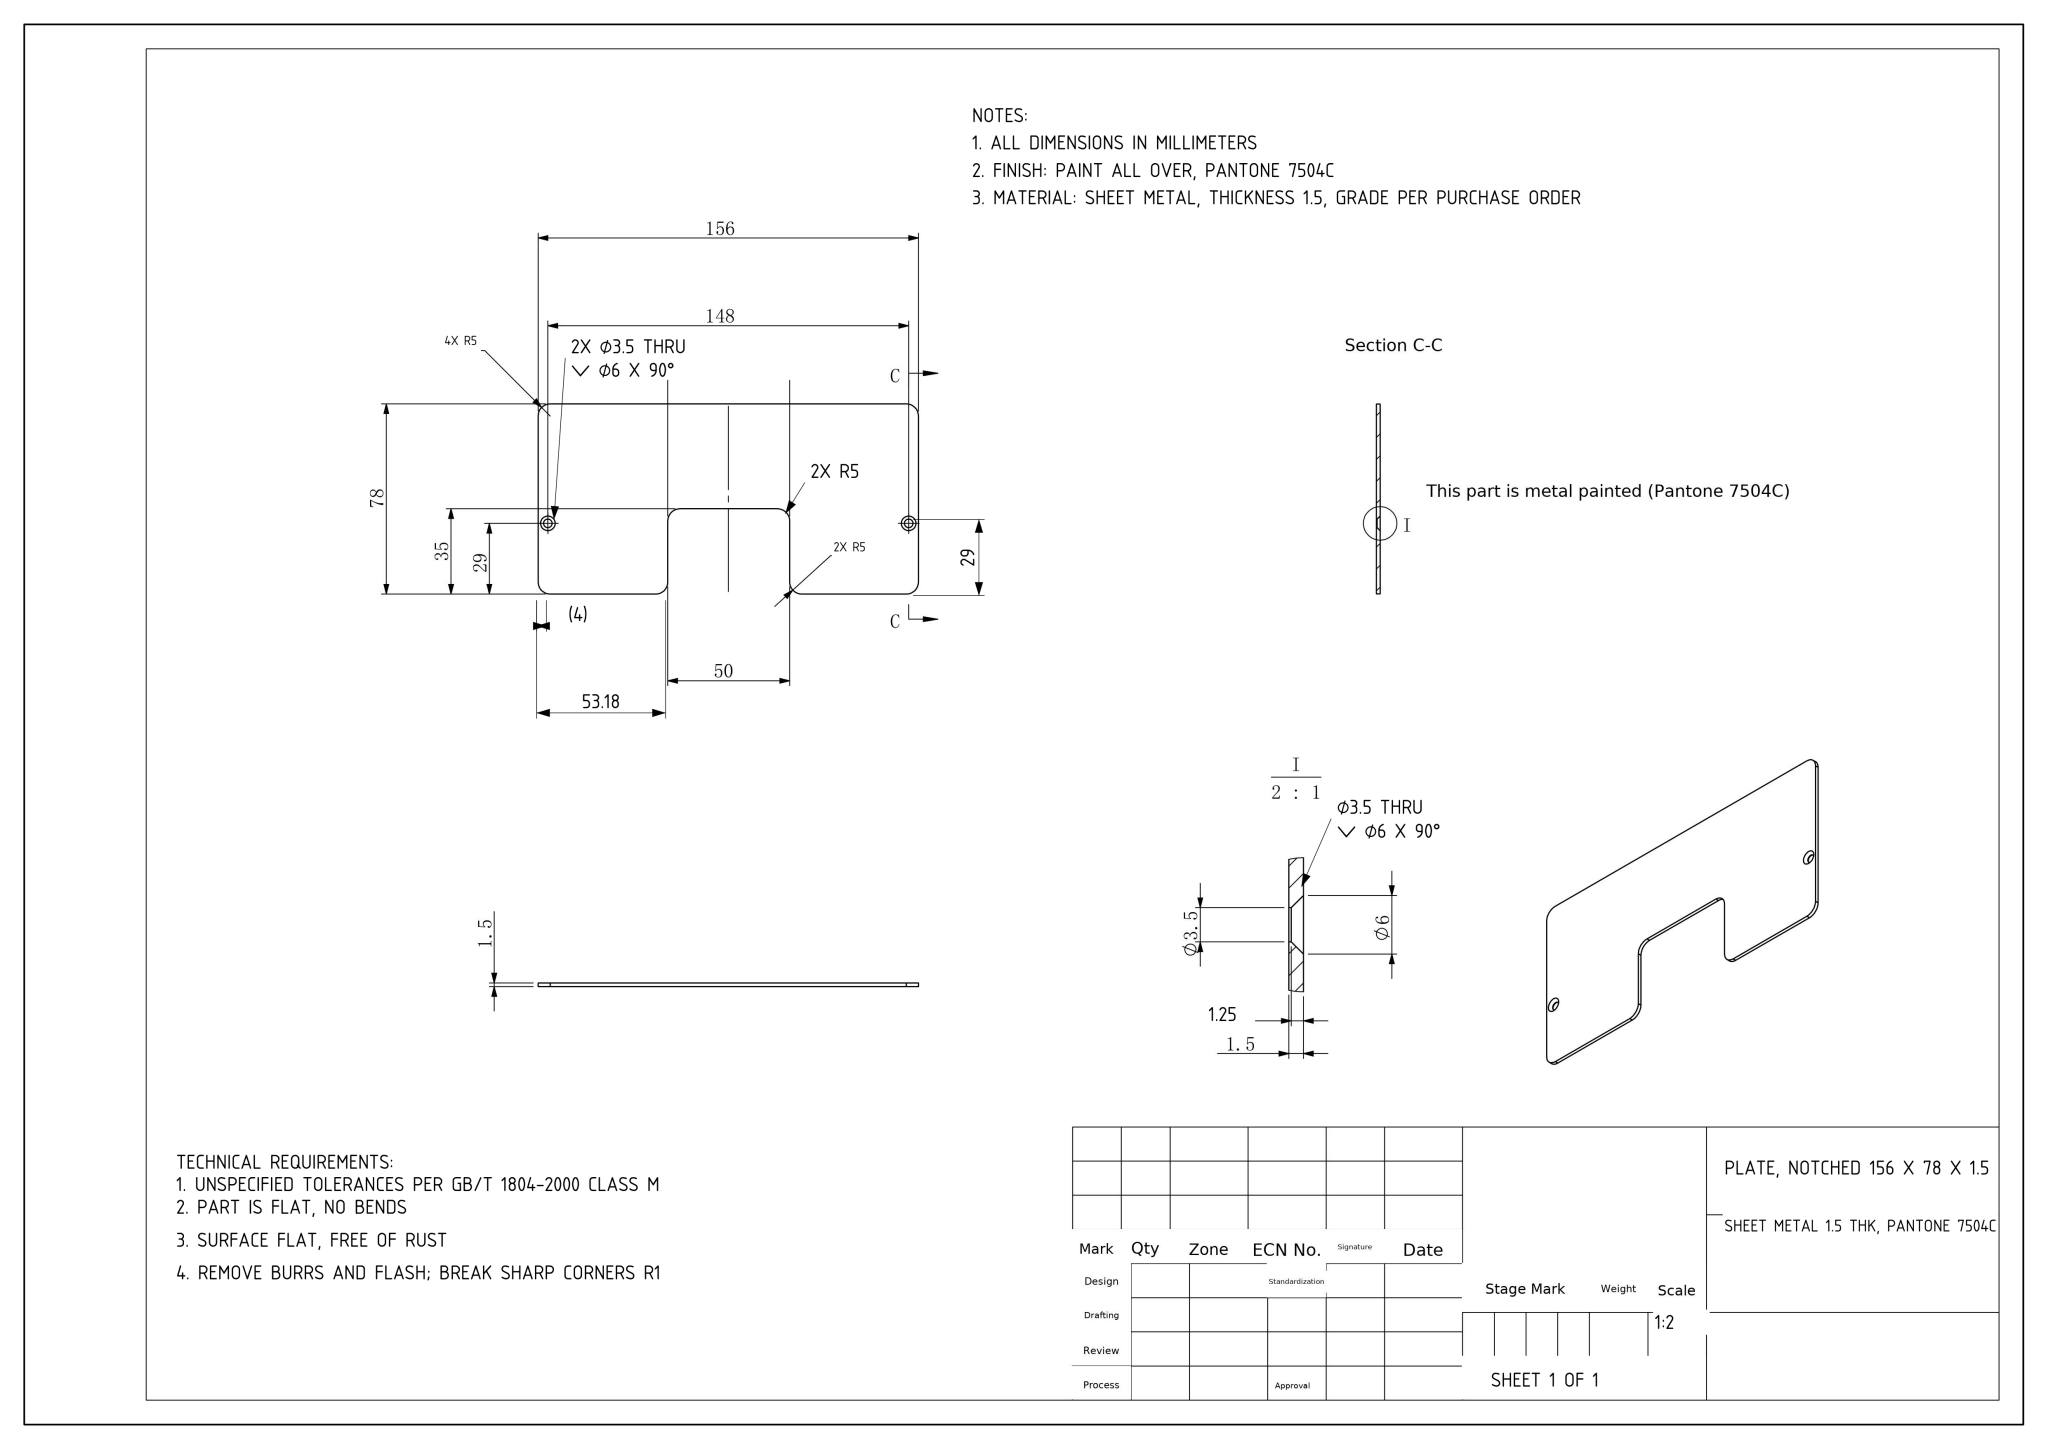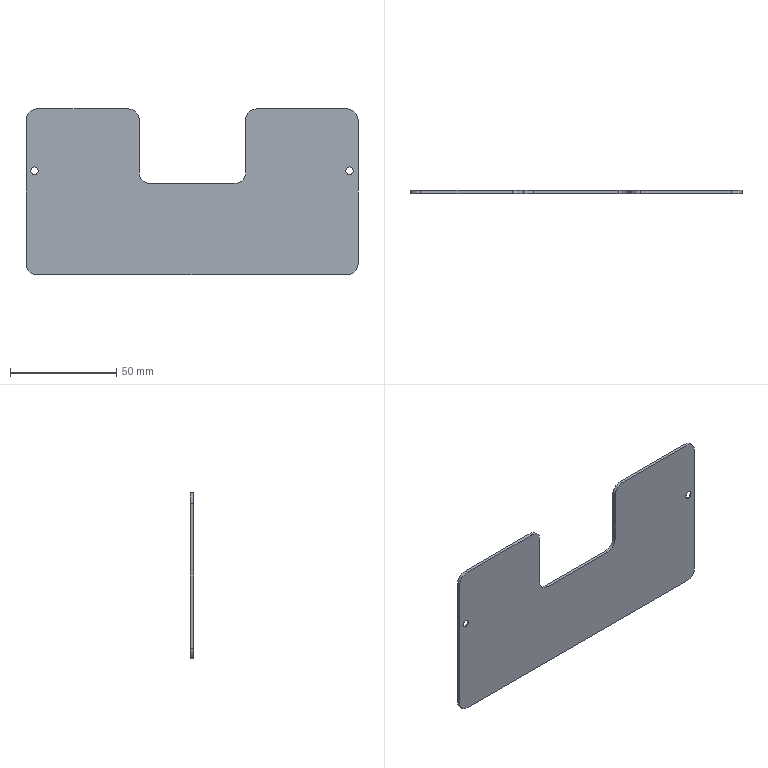Part | NX | mm | 1 solid | 26 faces | box 156 x 1.5 x 78 mm | volume 15545 mm3 | cylinder 12 | plane 10 | cone 4 | commonest cylinder face diameters 10 x8 3.5 x4
STEP:
#1=COLOUR_RGB('',0.7529,0.7529,0.7529);
#2=FILL_AREA_STYLE_COLOUR('',#1);
#3=FILL_AREA_STYLE('',(#2));
#4=SURFACE_STYLE_FILL_AREA(#3);
#5=SURFACE_SIDE_STYLE('',(#4));
#6=SURFACE_STYLE_USAGE(.BOTH.,#5);
#7=PRESENTATION_STYLE_ASSIGNMENT((#6));
#8=CARTESIAN_POINT('',(74.,-1.25,8.));
#9=VERTEX_POINT('',#8);
#10=CARTESIAN_POINT('',(74.,-1.25,11.5));
#11=VERTEX_POINT('',#10);
#12=CARTESIAN_POINT('',(74.,-1.25,9.75));
#13=DIRECTION('',(0.,1.,0.));
#14=DIRECTION('',(0.,0.,1.));
#15=AXIS2_PLACEMENT_3D('',#12,#13,#14);
#16=CIRCLE('',#15,1.75);
#17=EDGE_CURVE('',#9,#11,#16,.T.);
#18=ORIENTED_EDGE('',*,*,#17,.F.);
#19=CARTESIAN_POINT('',(74.,0.,6.75));
#20=VERTEX_POINT('',#19);
#21=CARTESIAN_POINT('',(74.,0.,6.75));
#22=DIRECTION('',(0.,0.7071,-0.7071));
#23=VECTOR('',#22,1000.);
#24=LINE('',#21,#23);
#25=EDGE_CURVE('',#9,#20,#24,.T.);
#26=ORIENTED_EDGE('',*,*,#25,.T.);
#27=CARTESIAN_POINT('',(74.,0.,12.75));
#28=VERTEX_POINT('',#27);
#29=CARTESIAN_POINT('',(74.,0.,9.75));
#30=DIRECTION('',(0.,-1.,0.));
#31=DIRECTION('',(0.,0.,1.));
#32=AXIS2_PLACEMENT_3D('',#29,#30,#31);
#33=CIRCLE('',#32,3.);
#34=EDGE_CURVE('',#28,#20,#33,.T.);
#35=ORIENTED_EDGE('',*,*,#34,.F.);
#36=CARTESIAN_POINT('',(74.,0.,12.75));
#37=DIRECTION('',(0.,0.7071,0.7071));
#38=VECTOR('',#37,1000.);
#39=LINE('',#36,#38);
#40=EDGE_CURVE('',#11,#28,#39,.T.);
#41=ORIENTED_EDGE('',*,*,#40,.F.);
#42=EDGE_LOOP('',(#18,#26,#35,#41));
#43=FACE_OUTER_BOUND('',#42,.T.);
#44=CARTESIAN_POINT('',(74.,0.,9.75));
#45=DIRECTION('',(0.,1.,0.));
#46=DIRECTION('',(0.,0.,1.));
#47=AXIS2_PLACEMENT_3D('',#44,#45,#46);
#48=CONICAL_SURFACE('',#47,3.,0.7854);
#49=ADVANCED_FACE('',(#43),#48,.F.);
#50=CARTESIAN_POINT('',(-74.,-1.25,8.));
#51=VERTEX_POINT('',#50);
#52=CARTESIAN_POINT('',(-74.,-1.25,11.5));
#53=VERTEX_POINT('',#52);
#54=CARTESIAN_POINT('',(-74.,-1.25,9.75));
#55=DIRECTION('',(0.,1.,0.));
#56=DIRECTION('',(0.,0.,1.));
#57=AXIS2_PLACEMENT_3D('',#54,#55,#56);
#58=CIRCLE('',#57,1.75);
#59=EDGE_CURVE('',#51,#53,#58,.T.);
#60=ORIENTED_EDGE('',*,*,#59,.F.);
#61=CARTESIAN_POINT('',(-74.,0.,6.75));
#62=VERTEX_POINT('',#61);
#63=CARTESIAN_POINT('',(-74.,0.,6.75));
#64=DIRECTION('',(0.,0.7071,-0.7071));
#65=VECTOR('',#64,1000.);
#66=LINE('',#63,#65);
#67=EDGE_CURVE('',#51,#62,#66,.T.);
#68=ORIENTED_EDGE('',*,*,#67,.T.);
#69=CARTESIAN_POINT('',(-74.,0.,12.75));
#70=VERTEX_POINT('',#69);
#71=CARTESIAN_POINT('',(-74.,0.,9.75));
#72=DIRECTION('',(0.,-1.,0.));
#73=DIRECTION('',(0.,0.,1.));
#74=AXIS2_PLACEMENT_3D('',#71,#72,#73);
#75=CIRCLE('',#74,3.);
#76=EDGE_CURVE('',#70,#62,#75,.T.);
#77=ORIENTED_EDGE('',*,*,#76,.F.);
#78=CARTESIAN_POINT('',(-74.,0.,12.75));
#79=DIRECTION('',(0.,0.7071,0.7071));
#80=VECTOR('',#79,1000.);
#81=LINE('',#78,#80);
#82=EDGE_CURVE('',#53,#70,#81,.T.);
#83=ORIENTED_EDGE('',*,*,#82,.F.);
#84=EDGE_LOOP('',(#60,#68,#77,#83));
#85=FACE_OUTER_BOUND('',#84,.T.);
#86=CARTESIAN_POINT('',(-74.,0.,9.75));
#87=DIRECTION('',(0.,1.,0.));
#88=DIRECTION('',(0.,0.,1.));
#89=AXIS2_PLACEMENT_3D('',#86,#87,#88);
#90=CONICAL_SURFACE('',#89,3.,0.7854);
#91=ADVANCED_FACE('',(#85),#90,.F.);
#92=ORIENTED_EDGE('',*,*,#17,.T.);
#93=CARTESIAN_POINT('',(74.,-1.5,11.5));
#94=VERTEX_POINT('',#93);
#95=CARTESIAN_POINT('',(74.,55.65,11.5));
#96=DIRECTION('',(0.,-1.,0.));
#97=VECTOR('',#96,1000.);
#98=LINE('',#95,#97);
#99=EDGE_CURVE('',#11,#94,#98,.T.);
#100=ORIENTED_EDGE('',*,*,#99,.T.);
#101=CARTESIAN_POINT('',(74.,-1.5,8.));
#102=VERTEX_POINT('',#101);
#103=CARTESIAN_POINT('',(74.,-1.5,9.75));
#104=DIRECTION('',(0.,1.,0.));
#105=DIRECTION('',(1.,0.,0.));
#106=AXIS2_PLACEMENT_3D('',#103,#104,#105);
#107=CIRCLE('',#106,1.75);
#108=EDGE_CURVE('',#102,#94,#107,.T.);
#109=ORIENTED_EDGE('',*,*,#108,.F.);
#110=CARTESIAN_POINT('',(74.,55.65,8.));
#111=DIRECTION('',(0.,-1.,0.));
#112=VECTOR('',#111,1000.);
#113=LINE('',#110,#112);
#114=EDGE_CURVE('',#9,#102,#113,.T.);
#115=ORIENTED_EDGE('',*,*,#114,.F.);
#116=EDGE_LOOP('',(#92,#100,#109,#115));
#117=FACE_OUTER_BOUND('',#116,.T.);
#118=CARTESIAN_POINT('',(74.,55.65,9.75));
#119=DIRECTION('',(0.,-1.,0.));
#120=DIRECTION('',(0.,0.,-1.));
#121=AXIS2_PLACEMENT_3D('',#118,#119,#120);
#122=CYLINDRICAL_SURFACE('',#121,1.75);
#123=ADVANCED_FACE('',(#117),#122,.F.);
#124=ORIENTED_EDGE('',*,*,#59,.T.);
#125=CARTESIAN_POINT('',(-74.,-1.5,11.5));
#126=VERTEX_POINT('',#125);
#127=CARTESIAN_POINT('',(-74.,55.65,11.5));
#128=DIRECTION('',(0.,-1.,0.));
#129=VECTOR('',#128,1000.);
#130=LINE('',#127,#129);
#131=EDGE_CURVE('',#53,#126,#130,.T.);
#132=ORIENTED_EDGE('',*,*,#131,.T.);
#133=CARTESIAN_POINT('',(-74.,-1.5,8.));
#134=VERTEX_POINT('',#133);
#135=CARTESIAN_POINT('',(-74.,-1.5,9.75));
#136=DIRECTION('',(0.,1.,0.));
#137=DIRECTION('',(1.,0.,0.));
#138=AXIS2_PLACEMENT_3D('',#135,#136,#137);
#139=CIRCLE('',#138,1.75);
#140=EDGE_CURVE('',#134,#126,#139,.T.);
#141=ORIENTED_EDGE('',*,*,#140,.F.);
#142=CARTESIAN_POINT('',(-74.,55.65,8.));
#143=DIRECTION('',(0.,-1.,0.));
#144=VECTOR('',#143,1000.);
#145=LINE('',#142,#144);
#146=EDGE_CURVE('',#51,#134,#145,.T.);
#147=ORIENTED_EDGE('',*,*,#146,.F.);
#148=EDGE_LOOP('',(#124,#132,#141,#147));
#149=FACE_OUTER_BOUND('',#148,.T.);
#150=CARTESIAN_POINT('',(-74.,55.65,9.75));
#151=DIRECTION('',(0.,-1.,0.));
#152=DIRECTION('',(0.,0.,-1.));
#153=AXIS2_PLACEMENT_3D('',#150,#151,#152);
#154=CYLINDRICAL_SURFACE('',#153,1.75);
#155=ADVANCED_FACE('',(#149),#154,.F.);
#156=CARTESIAN_POINT('',(30.185,0.,38.75));
#157=VERTEX_POINT('',#156);
#158=CARTESIAN_POINT('',(73.,0.,38.75));
#159=VERTEX_POINT('',#158);
#160=CARTESIAN_POINT('',(-78.5,0.,38.75));
#161=DIRECTION('',(1.,0.,0.));
#162=VECTOR('',#161,1000.);
#163=LINE('',#160,#162);
#164=EDGE_CURVE('',#157,#159,#163,.T.);
#165=ORIENTED_EDGE('',*,*,#164,.F.);
#166=CARTESIAN_POINT('',(30.185,-1.5,38.75));
#167=VERTEX_POINT('',#166);
#168=CARTESIAN_POINT('',(30.185,0.,38.75));
#169=DIRECTION('',(0.,-1.,0.));
#170=VECTOR('',#169,1000.);
#171=LINE('',#168,#170);
#172=EDGE_CURVE('',#157,#167,#171,.T.);
#173=ORIENTED_EDGE('',*,*,#172,.T.);
#174=CARTESIAN_POINT('',(73.,-1.5,38.75));
#175=VERTEX_POINT('',#174);
#176=CARTESIAN_POINT('',(-78.5,-1.5,38.75));
#177=DIRECTION('',(1.,0.,0.));
#178=VECTOR('',#177,1000.);
#179=LINE('',#176,#178);
#180=EDGE_CURVE('',#167,#175,#179,.T.);
#181=ORIENTED_EDGE('',*,*,#180,.T.);
#182=CARTESIAN_POINT('',(73.,0.,38.75));
#183=DIRECTION('',(0.,1.,0.));
#184=VECTOR('',#183,1000.);
#185=LINE('',#182,#184);
#186=EDGE_CURVE('',#175,#159,#185,.T.);
#187=ORIENTED_EDGE('',*,*,#186,.T.);
#188=EDGE_LOOP('',(#165,#173,#181,#187));
#189=FACE_OUTER_BOUND('',#188,.T.);
#190=CARTESIAN_POINT('',(-78.5,0.,38.75));
#191=DIRECTION('',(0.,0.,1.));
#192=DIRECTION('',(1.,0.,0.));
#193=AXIS2_PLACEMENT_3D('',#190,#191,#192);
#194=PLANE('',#193);
#195=ADVANCED_FACE('',(#189),#194,.T.);
#196=ORIENTED_EDGE('',*,*,#140,.T.);
#197=CARTESIAN_POINT('',(-74.,-1.5,9.75));
#198=DIRECTION('',(0.,1.,0.));
#199=DIRECTION('',(1.,0.,0.));
#200=AXIS2_PLACEMENT_3D('',#197,#198,#199);
#201=CIRCLE('',#200,1.75);
#202=EDGE_CURVE('',#126,#134,#201,.T.);
#203=ORIENTED_EDGE('',*,*,#202,.T.);
#204=EDGE_LOOP('',(#196,#203));
#205=FACE_BOUND('',#204,.T.);
#206=CARTESIAN_POINT('',(-24.815,-1.5,8.75));
#207=VERTEX_POINT('',#206);
#208=CARTESIAN_POINT('',(-24.815,-1.5,33.75));
#209=VERTEX_POINT('',#208);
#210=CARTESIAN_POINT('',(-24.815,-1.5,39.75));
#211=DIRECTION('',(0.,0.,1.));
#212=VECTOR('',#211,1000.);
#213=LINE('',#210,#212);
#214=EDGE_CURVE('',#207,#209,#213,.T.);
#215=ORIENTED_EDGE('',*,*,#214,.T.);
#216=CARTESIAN_POINT('',(-29.815,-1.5,38.75));
#217=VERTEX_POINT('',#216);
#218=CARTESIAN_POINT('',(-29.815,-1.5,33.75));
#219=DIRECTION('',(0.,-1.,0.));
#220=DIRECTION('',(0.,0.,1.));
#221=AXIS2_PLACEMENT_3D('',#218,#219,#220);
#222=CIRCLE('',#221,5.);
#223=EDGE_CURVE('',#209,#217,#222,.T.);
#224=ORIENTED_EDGE('',*,*,#223,.T.);
#225=CARTESIAN_POINT('',(-73.,-1.5,38.75));
#226=VERTEX_POINT('',#225);
#227=CARTESIAN_POINT('',(-78.5,-1.5,38.75));
#228=DIRECTION('',(1.,0.,0.));
#229=VECTOR('',#228,1000.);
#230=LINE('',#227,#229);
#231=EDGE_CURVE('',#226,#217,#230,.T.);
#232=ORIENTED_EDGE('',*,*,#231,.F.);
#233=CARTESIAN_POINT('',(-78.,-1.5,33.75));
#234=VERTEX_POINT('',#233);
#235=CARTESIAN_POINT('',(-73.,-1.5,33.75));
#236=DIRECTION('',(0.,-1.,0.));
#237=DIRECTION('',(0.,0.,1.));
#238=AXIS2_PLACEMENT_3D('',#235,#236,#237);
#239=CIRCLE('',#238,5.);
#240=EDGE_CURVE('',#226,#234,#239,.T.);
#241=ORIENTED_EDGE('',*,*,#240,.T.);
#242=CARTESIAN_POINT('',(-78.,-1.5,-34.25));
#243=VERTEX_POINT('',#242);
#244=CARTESIAN_POINT('',(-78.,-1.5,39.75));
#245=DIRECTION('',(0.,0.,1.));
#246=VECTOR('',#245,1000.);
#247=LINE('',#244,#246);
#248=EDGE_CURVE('',#243,#234,#247,.T.);
#249=ORIENTED_EDGE('',*,*,#248,.F.);
#250=CARTESIAN_POINT('',(-73.,-1.5,-39.25));
#251=VERTEX_POINT('',#250);
#252=CARTESIAN_POINT('',(-73.,-1.5,-34.25));
#253=DIRECTION('',(0.,1.,0.));
#254=DIRECTION('',(0.,0.,1.));
#255=AXIS2_PLACEMENT_3D('',#252,#253,#254);
#256=CIRCLE('',#255,5.);
#257=EDGE_CURVE('',#251,#243,#256,.T.);
#258=ORIENTED_EDGE('',*,*,#257,.F.);
#259=CARTESIAN_POINT('',(73.,-1.5,-39.25));
#260=VERTEX_POINT('',#259);
#261=CARTESIAN_POINT('',(-78.5,-1.5,-39.25));
#262=DIRECTION('',(-1.,0.,0.));
#263=VECTOR('',#262,1000.);
#264=LINE('',#261,#263);
#265=EDGE_CURVE('',#260,#251,#264,.T.);
#266=ORIENTED_EDGE('',*,*,#265,.F.);
#267=CARTESIAN_POINT('',(78.,-1.5,-34.25));
#268=VERTEX_POINT('',#267);
#269=CARTESIAN_POINT('',(73.,-1.5,-34.25));
#270=DIRECTION('',(0.,1.,0.));
#271=DIRECTION('',(0.,0.,1.));
#272=AXIS2_PLACEMENT_3D('',#269,#270,#271);
#273=CIRCLE('',#272,5.);
#274=EDGE_CURVE('',#268,#260,#273,.T.);
#275=ORIENTED_EDGE('',*,*,#274,.F.);
#276=CARTESIAN_POINT('',(78.,-1.5,33.75));
#277=VERTEX_POINT('',#276);
#278=CARTESIAN_POINT('',(78.,-1.5,39.75));
#279=DIRECTION('',(0.,0.,-1.));
#280=VECTOR('',#279,1000.);
#281=LINE('',#278,#280);
#282=EDGE_CURVE('',#277,#268,#281,.T.);
#283=ORIENTED_EDGE('',*,*,#282,.F.);
#284=CARTESIAN_POINT('',(73.,-1.5,33.75));
#285=DIRECTION('',(0.,-1.,0.));
#286=DIRECTION('',(0.,0.,1.));
#287=AXIS2_PLACEMENT_3D('',#284,#285,#286);
#288=CIRCLE('',#287,5.);
#289=EDGE_CURVE('',#277,#175,#288,.T.);
#290=ORIENTED_EDGE('',*,*,#289,.T.);
#291=ORIENTED_EDGE('',*,*,#180,.F.);
#292=CARTESIAN_POINT('',(25.185,-1.5,33.75));
#293=VERTEX_POINT('',#292);
#294=CARTESIAN_POINT('',(30.185,-1.5,33.75));
#295=DIRECTION('',(0.,-1.,0.));
#296=DIRECTION('',(0.,0.,1.));
#297=AXIS2_PLACEMENT_3D('',#294,#295,#296);
#298=CIRCLE('',#297,5.);
#299=EDGE_CURVE('',#167,#293,#298,.T.);
#300=ORIENTED_EDGE('',*,*,#299,.T.);
#301=CARTESIAN_POINT('',(25.185,-1.5,8.75));
#302=VERTEX_POINT('',#301);
#303=CARTESIAN_POINT('',(25.185,-1.5,39.75));
#304=DIRECTION('',(0.,0.,-1.));
#305=VECTOR('',#304,1000.);
#306=LINE('',#303,#305);
#307=EDGE_CURVE('',#293,#302,#306,.T.);
#308=ORIENTED_EDGE('',*,*,#307,.T.);
#309=CARTESIAN_POINT('',(20.185,-1.5,3.75));
#310=VERTEX_POINT('',#309);
#311=CARTESIAN_POINT('',(20.185,-1.5,8.75));
#312=DIRECTION('',(0.,1.,0.));
#313=DIRECTION('',(0.,0.,1.));
#314=AXIS2_PLACEMENT_3D('',#311,#312,#313);
#315=CIRCLE('',#314,5.);
#316=EDGE_CURVE('',#302,#310,#315,.T.);
#317=ORIENTED_EDGE('',*,*,#316,.T.);
#318=CARTESIAN_POINT('',(-19.815,-1.5,3.75));
#319=VERTEX_POINT('',#318);
#320=CARTESIAN_POINT('',(-78.5,-1.5,3.75));
#321=DIRECTION('',(-1.,0.,0.));
#322=VECTOR('',#321,1000.);
#323=LINE('',#320,#322);
#324=EDGE_CURVE('',#310,#319,#323,.T.);
#325=ORIENTED_EDGE('',*,*,#324,.T.);
#326=CARTESIAN_POINT('',(-19.815,-1.5,8.75));
#327=DIRECTION('',(0.,1.,0.));
#328=DIRECTION('',(0.,0.,1.));
#329=AXIS2_PLACEMENT_3D('',#326,#327,#328);
#330=CIRCLE('',#329,5.);
#331=EDGE_CURVE('',#319,#207,#330,.T.);
#332=ORIENTED_EDGE('',*,*,#331,.T.);
#333=EDGE_LOOP('',(#215,#224,#232,#241,#249,#258,#266,#275,#283,#290,#291,#300,#308,#317,#325,#332));
#334=FACE_OUTER_BOUND('',#333,.T.);
#335=ORIENTED_EDGE('',*,*,#108,.T.);
#336=CARTESIAN_POINT('',(74.,-1.5,9.75));
#337=DIRECTION('',(0.,1.,0.));
#338=DIRECTION('',(1.,0.,0.));
#339=AXIS2_PLACEMENT_3D('',#336,#337,#338);
#340=CIRCLE('',#339,1.75);
#341=EDGE_CURVE('',#94,#102,#340,.T.);
#342=ORIENTED_EDGE('',*,*,#341,.T.);
#343=EDGE_LOOP('',(#335,#342));
#344=FACE_BOUND('',#343,.T.);
#345=CARTESIAN_POINT('',(-78.5,-1.5,39.75));
#346=DIRECTION('',(0.,1.,0.));
#347=DIRECTION('',(0.,0.,1.));
#348=AXIS2_PLACEMENT_3D('',#345,#346,#347);
#349=PLANE('',#348);
#350=ADVANCED_FACE('',(#205,#334,#344),#349,.F.);
#351=CARTESIAN_POINT('',(-73.,0.,38.75));
#352=VERTEX_POINT('',#351);
#353=CARTESIAN_POINT('',(-29.815,0.,38.75));
#354=VERTEX_POINT('',#353);
#355=CARTESIAN_POINT('',(-78.5,0.,38.75));
#356=DIRECTION('',(1.,0.,0.));
#357=VECTOR('',#356,1000.);
#358=LINE('',#355,#357);
#359=EDGE_CURVE('',#352,#354,#358,.T.);
#360=ORIENTED_EDGE('',*,*,#359,.T.);
#361=CARTESIAN_POINT('',(-24.815,0.,33.75));
#362=VERTEX_POINT('',#361);
#363=CARTESIAN_POINT('',(-29.815,0.,33.75));
#364=DIRECTION('',(0.,1.,0.));
#365=DIRECTION('',(0.,0.,1.));
#366=AXIS2_PLACEMENT_3D('',#363,#364,#365);
#367=CIRCLE('',#366,5.);
#368=EDGE_CURVE('',#354,#362,#367,.T.);
#369=ORIENTED_EDGE('',*,*,#368,.T.);
#370=CARTESIAN_POINT('',(-24.815,0.,8.75));
#371=VERTEX_POINT('',#370);
#372=CARTESIAN_POINT('',(-24.815,0.,39.75));
#373=DIRECTION('',(0.,0.,1.));
#374=VECTOR('',#373,1000.);
#375=LINE('',#372,#374);
#376=EDGE_CURVE('',#371,#362,#375,.T.);
#377=ORIENTED_EDGE('',*,*,#376,.F.);
#378=CARTESIAN_POINT('',(-19.815,0.,3.75));
#379=VERTEX_POINT('',#378);
#380=CARTESIAN_POINT('',(-19.815,0.,8.75));
#381=DIRECTION('',(0.,-1.,0.));
#382=DIRECTION('',(0.,0.,1.));
#383=AXIS2_PLACEMENT_3D('',#380,#381,#382);
#384=CIRCLE('',#383,5.);
#385=EDGE_CURVE('',#371,#379,#384,.T.);
#386=ORIENTED_EDGE('',*,*,#385,.T.);
#387=CARTESIAN_POINT('',(20.185,0.,3.75));
#388=VERTEX_POINT('',#387);
#389=CARTESIAN_POINT('',(-78.5,0.,3.75));
#390=DIRECTION('',(-1.,0.,0.));
#391=VECTOR('',#390,1000.);
#392=LINE('',#389,#391);
#393=EDGE_CURVE('',#388,#379,#392,.T.);
#394=ORIENTED_EDGE('',*,*,#393,.F.);
#395=CARTESIAN_POINT('',(25.185,0.,8.75));
#396=VERTEX_POINT('',#395);
#397=CARTESIAN_POINT('',(20.185,0.,8.75));
#398=DIRECTION('',(0.,-1.,0.));
#399=DIRECTION('',(0.,0.,1.));
#400=AXIS2_PLACEMENT_3D('',#397,#398,#399);
#401=CIRCLE('',#400,5.);
#402=EDGE_CURVE('',#388,#396,#401,.T.);
#403=ORIENTED_EDGE('',*,*,#402,.T.);
#404=CARTESIAN_POINT('',(25.185,0.,33.75));
#405=VERTEX_POINT('',#404);
#406=CARTESIAN_POINT('',(25.185,0.,39.75));
#407=DIRECTION('',(0.,0.,-1.));
#408=VECTOR('',#407,1000.);
#409=LINE('',#406,#408);
#410=EDGE_CURVE('',#405,#396,#409,.T.);
#411=ORIENTED_EDGE('',*,*,#410,.F.);
#412=CARTESIAN_POINT('',(30.185,0.,33.75));
#413=DIRECTION('',(0.,1.,0.));
#414=DIRECTION('',(0.,0.,1.));
#415=AXIS2_PLACEMENT_3D('',#412,#413,#414);
#416=CIRCLE('',#415,5.);
#417=EDGE_CURVE('',#405,#157,#416,.T.);
#418=ORIENTED_EDGE('',*,*,#417,.T.);
#419=ORIENTED_EDGE('',*,*,#164,.T.);
#420=CARTESIAN_POINT('',(78.,0.,33.75));
#421=VERTEX_POINT('',#420);
#422=CARTESIAN_POINT('',(73.,0.,33.75));
#423=DIRECTION('',(0.,1.,0.));
#424=DIRECTION('',(0.,0.,1.));
#425=AXIS2_PLACEMENT_3D('',#422,#423,#424);
#426=CIRCLE('',#425,5.);
#427=EDGE_CURVE('',#159,#421,#426,.T.);
#428=ORIENTED_EDGE('',*,*,#427,.T.);
#429=CARTESIAN_POINT('',(78.,0.,-34.25));
#430=VERTEX_POINT('',#429);
#431=CARTESIAN_POINT('',(78.,0.,39.75));
#432=DIRECTION('',(0.,0.,-1.));
#433=VECTOR('',#432,1000.);
#434=LINE('',#431,#433);
#435=EDGE_CURVE('',#421,#430,#434,.T.);
#436=ORIENTED_EDGE('',*,*,#435,.T.);
#437=CARTESIAN_POINT('',(73.,0.,-39.25));
#438=VERTEX_POINT('',#437);
#439=CARTESIAN_POINT('',(73.,0.,-34.25));
#440=DIRECTION('',(0.,1.,0.));
#441=DIRECTION('',(0.,0.,1.));
#442=AXIS2_PLACEMENT_3D('',#439,#440,#441);
#443=CIRCLE('',#442,5.);
#444=EDGE_CURVE('',#430,#438,#443,.T.);
#445=ORIENTED_EDGE('',*,*,#444,.T.);
#446=CARTESIAN_POINT('',(-73.,0.,-39.25));
#447=VERTEX_POINT('',#446);
#448=CARTESIAN_POINT('',(-78.5,0.,-39.25));
#449=DIRECTION('',(-1.,0.,-0.));
#450=VECTOR('',#449,1000.);
#451=LINE('',#448,#450);
#452=EDGE_CURVE('',#438,#447,#451,.T.);
#453=ORIENTED_EDGE('',*,*,#452,.T.);
#454=CARTESIAN_POINT('',(-78.,0.,-34.25));
#455=VERTEX_POINT('',#454);
#456=CARTESIAN_POINT('',(-73.,0.,-34.25));
#457=DIRECTION('',(0.,1.,0.));
#458=DIRECTION('',(0.,0.,1.));
#459=AXIS2_PLACEMENT_3D('',#456,#457,#458);
#460=CIRCLE('',#459,5.);
#461=EDGE_CURVE('',#447,#455,#460,.T.);
#462=ORIENTED_EDGE('',*,*,#461,.T.);
#463=CARTESIAN_POINT('',(-78.,0.,33.75));
#464=VERTEX_POINT('',#463);
#465=CARTESIAN_POINT('',(-78.,0.,39.75));
#466=DIRECTION('',(0.,0.,1.));
#467=VECTOR('',#466,1000.);
#468=LINE('',#465,#467);
#469=EDGE_CURVE('',#455,#464,#468,.T.);
#470=ORIENTED_EDGE('',*,*,#469,.T.);
#471=CARTESIAN_POINT('',(-73.,0.,33.75));
#472=DIRECTION('',(0.,1.,0.));
#473=DIRECTION('',(0.,0.,1.));
#474=AXIS2_PLACEMENT_3D('',#471,#472,#473);
#475=CIRCLE('',#474,5.);
#476=EDGE_CURVE('',#464,#352,#475,.T.);
#477=ORIENTED_EDGE('',*,*,#476,.T.);
#478=EDGE_LOOP('',(#360,#369,#377,#386,#394,#403,#411,#418,#419,#428,#436,#445,#453,#462,#470,#477));
#479=FACE_OUTER_BOUND('',#478,.T.);
#480=ORIENTED_EDGE('',*,*,#76,.T.);
#481=CARTESIAN_POINT('',(-74.,0.,9.75));
#482=DIRECTION('',(0.,-1.,0.));
#483=DIRECTION('',(0.,0.,1.));
#484=AXIS2_PLACEMENT_3D('',#481,#482,#483);
#485=CIRCLE('',#484,3.);
#486=EDGE_CURVE('',#62,#70,#485,.T.);
#487=ORIENTED_EDGE('',*,*,#486,.T.);
#488=EDGE_LOOP('',(#480,#487));
#489=FACE_BOUND('',#488,.T.);
#490=ORIENTED_EDGE('',*,*,#34,.T.);
#491=CARTESIAN_POINT('',(74.,0.,9.75));
#492=DIRECTION('',(0.,-1.,0.));
#493=DIRECTION('',(0.,0.,1.));
#494=AXIS2_PLACEMENT_3D('',#491,#492,#493);
#495=CIRCLE('',#494,3.);
#496=EDGE_CURVE('',#20,#28,#495,.T.);
#497=ORIENTED_EDGE('',*,*,#496,.T.);
#498=EDGE_LOOP('',(#490,#497));
#499=FACE_BOUND('',#498,.T.);
#500=CARTESIAN_POINT('',(-78.5,0.,39.75));
#501=DIRECTION('',(0.,1.,0.));
#502=DIRECTION('',(0.,0.,1.));
#503=AXIS2_PLACEMENT_3D('',#500,#501,#502);
#504=PLANE('',#503);
#505=ADVANCED_FACE('',(#479,#489,#499),#504,.T.);
#506=ORIENTED_EDGE('',*,*,#131,.F.);
#507=CARTESIAN_POINT('',(-74.,-1.25,9.75));
#508=DIRECTION('',(0.,1.,0.));
#509=DIRECTION('',(0.,0.,1.));
#510=AXIS2_PLACEMENT_3D('',#507,#508,#509);
#511=CIRCLE('',#510,1.75);
#512=EDGE_CURVE('',#53,#51,#511,.T.);
#513=ORIENTED_EDGE('',*,*,#512,.T.);
#514=ORIENTED_EDGE('',*,*,#146,.T.);
#515=ORIENTED_EDGE('',*,*,#202,.F.);
#516=EDGE_LOOP('',(#506,#513,#514,#515));
#517=FACE_OUTER_BOUND('',#516,.T.);
#518=CARTESIAN_POINT('',(-74.,55.65,9.75));
#519=DIRECTION('',(0.,-1.,0.));
#520=DIRECTION('',(0.,0.,-1.));
#521=AXIS2_PLACEMENT_3D('',#518,#519,#520);
#522=CYLINDRICAL_SURFACE('',#521,1.75);
#523=ADVANCED_FACE('',(#517),#522,.F.);
#524=ORIENTED_EDGE('',*,*,#99,.F.);
#525=CARTESIAN_POINT('',(74.,-1.25,9.75));
#526=DIRECTION('',(0.,1.,0.));
#527=DIRECTION('',(0.,0.,1.));
#528=AXIS2_PLACEMENT_3D('',#525,#526,#527);
#529=CIRCLE('',#528,1.75);
#530=EDGE_CURVE('',#11,#9,#529,.T.);
#531=ORIENTED_EDGE('',*,*,#530,.T.);
#532=ORIENTED_EDGE('',*,*,#114,.T.);
#533=ORIENTED_EDGE('',*,*,#341,.F.);
#534=EDGE_LOOP('',(#524,#531,#532,#533));
#535=FACE_OUTER_BOUND('',#534,.T.);
#536=CARTESIAN_POINT('',(74.,55.65,9.75));
#537=DIRECTION('',(0.,-1.,0.));
#538=DIRECTION('',(0.,0.,-1.));
#539=AXIS2_PLACEMENT_3D('',#536,#537,#538);
#540=CYLINDRICAL_SURFACE('',#539,1.75);
#541=ADVANCED_FACE('',(#535),#540,.F.);
#542=ORIENTED_EDGE('',*,*,#67,.F.);
#543=ORIENTED_EDGE('',*,*,#512,.F.);
#544=ORIENTED_EDGE('',*,*,#82,.T.);
#545=ORIENTED_EDGE('',*,*,#486,.F.);
#546=EDGE_LOOP('',(#542,#543,#544,#545));
#547=FACE_OUTER_BOUND('',#546,.T.);
#548=CARTESIAN_POINT('',(-74.,0.,9.75));
#549=DIRECTION('',(0.,1.,0.));
#550=DIRECTION('',(0.,0.,1.));
#551=AXIS2_PLACEMENT_3D('',#548,#549,#550);
#552=CONICAL_SURFACE('',#551,3.,0.7854);
#553=ADVANCED_FACE('',(#547),#552,.F.);
#554=ORIENTED_EDGE('',*,*,#25,.F.);
#555=ORIENTED_EDGE('',*,*,#530,.F.);
#556=ORIENTED_EDGE('',*,*,#40,.T.);
#557=ORIENTED_EDGE('',*,*,#496,.F.);
#558=EDGE_LOOP('',(#554,#555,#556,#557));
#559=FACE_OUTER_BOUND('',#558,.T.);
#560=CARTESIAN_POINT('',(74.,0.,9.75));
#561=DIRECTION('',(0.,1.,0.));
#562=DIRECTION('',(0.,0.,1.));
#563=AXIS2_PLACEMENT_3D('',#560,#561,#562);
#564=CONICAL_SURFACE('',#563,3.,0.7854);
#565=ADVANCED_FACE('',(#559),#564,.F.);
#566=ORIENTED_EDGE('',*,*,#231,.T.);
#567=CARTESIAN_POINT('',(-29.815,0.,38.75));
#568=DIRECTION('',(0.,1.,0.));
#569=VECTOR('',#568,1000.);
#570=LINE('',#567,#569);
#571=EDGE_CURVE('',#217,#354,#570,.T.);
#572=ORIENTED_EDGE('',*,*,#571,.T.);
#573=ORIENTED_EDGE('',*,*,#359,.F.);
#574=CARTESIAN_POINT('',(-73.,0.,38.75));
#575=DIRECTION('',(0.,-1.,0.));
#576=VECTOR('',#575,1000.);
#577=LINE('',#574,#576);
#578=EDGE_CURVE('',#352,#226,#577,.T.);
#579=ORIENTED_EDGE('',*,*,#578,.T.);
#580=EDGE_LOOP('',(#566,#572,#573,#579));
#581=FACE_OUTER_BOUND('',#580,.T.);
#582=CARTESIAN_POINT('',(-78.5,0.,38.75));
#583=DIRECTION('',(0.,0.,1.));
#584=DIRECTION('',(1.,0.,0.));
#585=AXIS2_PLACEMENT_3D('',#582,#583,#584);
#586=PLANE('',#585);
#587=ADVANCED_FACE('',(#581),#586,.T.);
#588=ORIENTED_EDGE('',*,*,#248,.T.);
#589=CARTESIAN_POINT('',(-78.,0.,33.75));
#590=DIRECTION('',(0.,1.,0.));
#591=VECTOR('',#590,1000.);
#592=LINE('',#589,#591);
#593=EDGE_CURVE('',#234,#464,#592,.T.);
#594=ORIENTED_EDGE('',*,*,#593,.T.);
#595=ORIENTED_EDGE('',*,*,#469,.F.);
#596=CARTESIAN_POINT('',(-78.,0.,-34.25));
#597=DIRECTION('',(0.,1.,0.));
#598=VECTOR('',#597,1000.);
#599=LINE('',#596,#598);
#600=EDGE_CURVE('',#243,#455,#599,.T.);
#601=ORIENTED_EDGE('',*,*,#600,.F.);
#602=EDGE_LOOP('',(#588,#594,#595,#601));
#603=FACE_OUTER_BOUND('',#602,.T.);
#604=CARTESIAN_POINT('',(-78.,0.,39.75));
#605=DIRECTION('',(-1.,0.,0.));
#606=DIRECTION('',(0.,0.,1.));
#607=AXIS2_PLACEMENT_3D('',#604,#605,#606);
#608=PLANE('',#607);
#609=ADVANCED_FACE('',(#603),#608,.T.);
#610=ORIENTED_EDGE('',*,*,#600,.T.);
#611=ORIENTED_EDGE('',*,*,#461,.F.);
#612=CARTESIAN_POINT('',(-73.,0.,-39.25));
#613=DIRECTION('',(0.,1.,0.));
#614=VECTOR('',#613,1000.);
#615=LINE('',#612,#614);
#616=EDGE_CURVE('',#251,#447,#615,.T.);
#617=ORIENTED_EDGE('',*,*,#616,.F.);
#618=ORIENTED_EDGE('',*,*,#257,.T.);
#619=EDGE_LOOP('',(#610,#611,#617,#618));
#620=FACE_OUTER_BOUND('',#619,.T.);
#621=CARTESIAN_POINT('',(-73.,0.,-34.25));
#622=DIRECTION('',(0.,1.,0.));
#623=DIRECTION('',(0.,0.,1.));
#624=AXIS2_PLACEMENT_3D('',#621,#622,#623);
#625=CYLINDRICAL_SURFACE('',#624,5.);
#626=ADVANCED_FACE('',(#620),#625,.T.);
#627=ORIENTED_EDGE('',*,*,#616,.T.);
#628=ORIENTED_EDGE('',*,*,#452,.F.);
#629=CARTESIAN_POINT('',(73.,0.,-39.25));
#630=DIRECTION('',(0.,1.,0.));
#631=VECTOR('',#630,1000.);
#632=LINE('',#629,#631);
#633=EDGE_CURVE('',#260,#438,#632,.T.);
#634=ORIENTED_EDGE('',*,*,#633,.F.);
#635=ORIENTED_EDGE('',*,*,#265,.T.);
#636=EDGE_LOOP('',(#627,#628,#634,#635));
#637=FACE_OUTER_BOUND('',#636,.T.);
#638=CARTESIAN_POINT('',(-78.5,0.,-39.25));
#639=DIRECTION('',(0.,0.,-1.));
#640=DIRECTION('',(-1.,0.,-0.));
#641=AXIS2_PLACEMENT_3D('',#638,#639,#640);
#642=PLANE('',#641);
#643=ADVANCED_FACE('',(#637),#642,.T.);
#644=ORIENTED_EDGE('',*,*,#633,.T.);
#645=ORIENTED_EDGE('',*,*,#444,.F.);
#646=CARTESIAN_POINT('',(78.,0.,-34.25));
#647=DIRECTION('',(0.,1.,0.));
#648=VECTOR('',#647,1000.);
#649=LINE('',#646,#648);
#650=EDGE_CURVE('',#268,#430,#649,.T.);
#651=ORIENTED_EDGE('',*,*,#650,.F.);
#652=ORIENTED_EDGE('',*,*,#274,.T.);
#653=EDGE_LOOP('',(#644,#645,#651,#652));
#654=FACE_OUTER_BOUND('',#653,.T.);
#655=CARTESIAN_POINT('',(73.,0.,-34.25));
#656=DIRECTION('',(0.,1.,0.));
#657=DIRECTION('',(0.,0.,1.));
#658=AXIS2_PLACEMENT_3D('',#655,#656,#657);
#659=CYLINDRICAL_SURFACE('',#658,5.);
#660=ADVANCED_FACE('',(#654),#659,.T.);
#661=ORIENTED_EDGE('',*,*,#435,.F.);
#662=CARTESIAN_POINT('',(78.,0.,33.75));
#663=DIRECTION('',(0.,-1.,0.));
#664=VECTOR('',#663,1000.);
#665=LINE('',#662,#664);
#666=EDGE_CURVE('',#421,#277,#665,.T.);
#667=ORIENTED_EDGE('',*,*,#666,.T.);
#668=ORIENTED_EDGE('',*,*,#282,.T.);
#669=ORIENTED_EDGE('',*,*,#650,.T.);
#670=EDGE_LOOP('',(#661,#667,#668,#669));
#671=FACE_OUTER_BOUND('',#670,.T.);
#672=CARTESIAN_POINT('',(78.,0.,39.75));
#673=DIRECTION('',(1.,0.,0.));
#674=DIRECTION('',(0.,0.,-1.));
#675=AXIS2_PLACEMENT_3D('',#672,#673,#674);
#676=PLANE('',#675);
#677=ADVANCED_FACE('',(#671),#676,.T.);
#678=ORIENTED_EDGE('',*,*,#240,.F.);
#679=ORIENTED_EDGE('',*,*,#578,.F.);
#680=ORIENTED_EDGE('',*,*,#476,.F.);
#681=ORIENTED_EDGE('',*,*,#593,.F.);
#682=EDGE_LOOP('',(#678,#679,#680,#681));
#683=FACE_OUTER_BOUND('',#682,.T.);
#684=CARTESIAN_POINT('',(-73.,0.,33.75));
#685=DIRECTION('',(0.,1.,0.));
#686=DIRECTION('',(0.,0.,1.));
#687=AXIS2_PLACEMENT_3D('',#684,#685,#686);
#688=CYLINDRICAL_SURFACE('',#687,5.);
#689=ADVANCED_FACE('',(#683),#688,.T.);
#690=ORIENTED_EDGE('',*,*,#289,.F.);
#691=ORIENTED_EDGE('',*,*,#666,.F.);
#692=ORIENTED_EDGE('',*,*,#427,.F.);
#693=ORIENTED_EDGE('',*,*,#186,.F.);
#694=EDGE_LOOP('',(#690,#691,#692,#693));
#695=FACE_OUTER_BOUND('',#694,.T.);
#696=CARTESIAN_POINT('',(73.,0.,33.75));
#697=DIRECTION('',(0.,1.,0.));
#698=DIRECTION('',(0.,0.,1.));
#699=AXIS2_PLACEMENT_3D('',#696,#697,#698);
#700=CYLINDRICAL_SURFACE('',#699,5.);
#701=ADVANCED_FACE('',(#695),#700,.T.);
#702=ORIENTED_EDGE('',*,*,#307,.F.);
#703=CARTESIAN_POINT('',(25.185,0.,33.75));
#704=DIRECTION('',(0.,1.,0.));
#705=VECTOR('',#704,1000.);
#706=LINE('',#703,#705);
#707=EDGE_CURVE('',#293,#405,#706,.T.);
#708=ORIENTED_EDGE('',*,*,#707,.T.);
#709=ORIENTED_EDGE('',*,*,#410,.T.);
#710=CARTESIAN_POINT('',(25.185,-1.5,8.75));
#711=DIRECTION('',(0.,-1.,0.));
#712=VECTOR('',#711,1000.);
#713=LINE('',#710,#712);
#714=EDGE_CURVE('',#396,#302,#713,.T.);
#715=ORIENTED_EDGE('',*,*,#714,.T.);
#716=EDGE_LOOP('',(#702,#708,#709,#715));
#717=FACE_OUTER_BOUND('',#716,.T.);
#718=CARTESIAN_POINT('',(25.185,0.,39.75));
#719=DIRECTION('',(1.,0.,0.));
#720=DIRECTION('',(0.,0.,-1.));
#721=AXIS2_PLACEMENT_3D('',#718,#719,#720);
#722=PLANE('',#721);
#723=ADVANCED_FACE('',(#717),#722,.F.);
#724=ORIENTED_EDGE('',*,*,#324,.F.);
#725=CARTESIAN_POINT('',(20.185,0.,3.75));
#726=DIRECTION('',(0.,1.,0.));
#727=VECTOR('',#726,1000.);
#728=LINE('',#725,#727);
#729=EDGE_CURVE('',#310,#388,#728,.T.);
#730=ORIENTED_EDGE('',*,*,#729,.T.);
#731=ORIENTED_EDGE('',*,*,#393,.T.);
#732=CARTESIAN_POINT('',(-19.815,-1.5,3.75));
#733=DIRECTION('',(0.,-1.,0.));
#734=VECTOR('',#733,1000.);
#735=LINE('',#732,#734);
#736=EDGE_CURVE('',#379,#319,#735,.T.);
#737=ORIENTED_EDGE('',*,*,#736,.T.);
#738=EDGE_LOOP('',(#724,#730,#731,#737));
#739=FACE_OUTER_BOUND('',#738,.T.);
#740=CARTESIAN_POINT('',(-78.5,0.,3.75));
#741=DIRECTION('',(0.,0.,-1.));
#742=DIRECTION('',(-1.,0.,0.));
#743=AXIS2_PLACEMENT_3D('',#740,#741,#742);
#744=PLANE('',#743);
#745=ADVANCED_FACE('',(#739),#744,.F.);
#746=ORIENTED_EDGE('',*,*,#376,.T.);
#747=CARTESIAN_POINT('',(-24.815,0.,33.75));
#748=DIRECTION('',(0.,-1.,0.));
#749=VECTOR('',#748,1000.);
#750=LINE('',#747,#749);
#751=EDGE_CURVE('',#362,#209,#750,.T.);
#752=ORIENTED_EDGE('',*,*,#751,.T.);
#753=ORIENTED_EDGE('',*,*,#214,.F.);
#754=CARTESIAN_POINT('',(-24.815,0.,8.75));
#755=DIRECTION('',(0.,1.,0.));
#756=VECTOR('',#755,1000.);
#757=LINE('',#754,#756);
#758=EDGE_CURVE('',#207,#371,#757,.T.);
#759=ORIENTED_EDGE('',*,*,#758,.T.);
#760=EDGE_LOOP('',(#746,#752,#753,#759));
#761=FACE_OUTER_BOUND('',#760,.T.);
#762=CARTESIAN_POINT('',(-24.815,0.,39.75));
#763=DIRECTION('',(-1.,0.,0.));
#764=DIRECTION('',(0.,0.,1.));
#765=AXIS2_PLACEMENT_3D('',#762,#763,#764);
#766=PLANE('',#765);
#767=ADVANCED_FACE('',(#761),#766,.F.);
#768=ORIENTED_EDGE('',*,*,#223,.F.);
#769=ORIENTED_EDGE('',*,*,#751,.F.);
#770=ORIENTED_EDGE('',*,*,#368,.F.);
#771=ORIENTED_EDGE('',*,*,#571,.F.);
#772=EDGE_LOOP('',(#768,#769,#770,#771));
#773=FACE_OUTER_BOUND('',#772,.T.);
#774=CARTESIAN_POINT('',(-29.815,0.,33.75));
#775=DIRECTION('',(0.,-1.,0.));
#776=DIRECTION('',(0.,0.,-1.));
#777=AXIS2_PLACEMENT_3D('',#774,#775,#776);
#778=CYLINDRICAL_SURFACE('',#777,5.);
#779=ADVANCED_FACE('',(#773),#778,.T.);
#780=ORIENTED_EDGE('',*,*,#299,.F.);
#781=ORIENTED_EDGE('',*,*,#172,.F.);
#782=ORIENTED_EDGE('',*,*,#417,.F.);
#783=ORIENTED_EDGE('',*,*,#707,.F.);
#784=EDGE_LOOP('',(#780,#781,#782,#783));
#785=FACE_OUTER_BOUND('',#784,.T.);
#786=CARTESIAN_POINT('',(30.185,0.,33.75));
#787=DIRECTION('',(0.,-1.,0.));
#788=DIRECTION('',(0.,0.,-1.));
#789=AXIS2_PLACEMENT_3D('',#786,#787,#788);
#790=CYLINDRICAL_SURFACE('',#789,5.);
#791=ADVANCED_FACE('',(#785),#790,.T.);
#792=ORIENTED_EDGE('',*,*,#316,.F.);
#793=ORIENTED_EDGE('',*,*,#714,.F.);
#794=ORIENTED_EDGE('',*,*,#402,.F.);
#795=ORIENTED_EDGE('',*,*,#729,.F.);
#796=EDGE_LOOP('',(#792,#793,#794,#795));
#797=FACE_OUTER_BOUND('',#796,.T.);
#798=CARTESIAN_POINT('',(20.185,0.,8.75));
#799=DIRECTION('',(0.,-1.,0.));
#800=DIRECTION('',(0.,0.,-1.));
#801=AXIS2_PLACEMENT_3D('',#798,#799,#800);
#802=CYLINDRICAL_SURFACE('',#801,5.);
#803=ADVANCED_FACE('',(#797),#802,.F.);
#804=ORIENTED_EDGE('',*,*,#331,.F.);
#805=ORIENTED_EDGE('',*,*,#736,.F.);
#806=ORIENTED_EDGE('',*,*,#385,.F.);
#807=ORIENTED_EDGE('',*,*,#758,.F.);
#808=EDGE_LOOP('',(#804,#805,#806,#807));
#809=FACE_OUTER_BOUND('',#808,.T.);
#810=CARTESIAN_POINT('',(-19.815,0.,8.75));
#811=DIRECTION('',(0.,-1.,0.));
#812=DIRECTION('',(0.,0.,-1.));
#813=AXIS2_PLACEMENT_3D('',#810,#811,#812);
#814=CYLINDRICAL_SURFACE('',#813,5.);
#815=ADVANCED_FACE('',(#809),#814,.F.);
#816=CLOSED_SHELL('',(#49,#91,#123,#155,#195,#350,#505,#523,#541,#553,#565,#587,#609,#626,#643,#660,#677,#689,#701,#723,#745,#767,#779,#791,#803,#815));
#817=MANIFOLD_SOLID_BREP('',#816);
#818=CARTESIAN_POINT('',(0.,0.,0.));
#819=DIRECTION('',(0.,0.,1.));
#820=DIRECTION('',(1.,0.,0.));
#821=AXIS2_PLACEMENT_3D('',#818,#819,#820);
#822=(LENGTH_UNIT()NAMED_UNIT(*)SI_UNIT(.MILLI.,.METRE.));
#823=UNCERTAINTY_MEASURE_WITH_UNIT(LENGTH_MEASURE(0.00001),#822,'','');
#824=(NAMED_UNIT(*)PLANE_ANGLE_UNIT()SI_UNIT($,.RADIAN.));
#825=(NAMED_UNIT(*)SI_UNIT($,.STERADIAN.)SOLID_ANGLE_UNIT());
#826=(GEOMETRIC_REPRESENTATION_CONTEXT(3)GLOBAL_UNCERTAINTY_ASSIGNED_CONTEXT((#823))GLOBAL_UNIT_ASSIGNED_CONTEXT((#822,#824,#825))REPRESENTATION_CONTEXT('',''));
#827=ADVANCED_BREP_SHAPE_REPRESENTATION('',(#817,#821),#826);
#828=STYLED_ITEM('',(#7),#827);
#829=(LENGTH_UNIT()NAMED_UNIT(*)SI_UNIT(.MILLI.,.METRE.));
#830=UNCERTAINTY_MEASURE_WITH_UNIT(LENGTH_MEASURE(0.00001),#829,'','');
#831=(NAMED_UNIT(*)PLANE_ANGLE_UNIT()SI_UNIT($,.RADIAN.));
#832=(NAMED_UNIT(*)SI_UNIT($,.STERADIAN.)SOLID_ANGLE_UNIT());
#833=(GEOMETRIC_REPRESENTATION_CONTEXT(3)GLOBAL_UNCERTAINTY_ASSIGNED_CONTEXT((#830))GLOBAL_UNIT_ASSIGNED_CONTEXT((#829,#831,#832))REPRESENTATION_CONTEXT('',''));
#834=MECHANICAL_DESIGN_GEOMETRIC_PRESENTATION_REPRESENTATION('',(#828),#833);
#835=PRESENTATION_LAYER_ASSIGNMENT('','',(#828));
#836=COLOUR_RGB('',0.7529,0.7529,0.7529);
#837=FILL_AREA_STYLE_COLOUR('',#836);
#838=FILL_AREA_STYLE('',(#837));
#839=SURFACE_STYLE_FILL_AREA(#838);
#840=SURFACE_SIDE_STYLE('',(#839));
#841=SURFACE_STYLE_USAGE(.BOTH.,#840);
#842=PRESENTATION_STYLE_ASSIGNMENT((#841));
#843=STYLED_ITEM('',(#842),#817);
#844=(LENGTH_UNIT()NAMED_UNIT(*)SI_UNIT(.MILLI.,.METRE.));
#845=UNCERTAINTY_MEASURE_WITH_UNIT(LENGTH_MEASURE(0.00001),#844,'','');
#846=(NAMED_UNIT(*)PLANE_ANGLE_UNIT()SI_UNIT($,.RADIAN.));
#847=(NAMED_UNIT(*)SI_UNIT($,.STERADIAN.)SOLID_ANGLE_UNIT());
#848=(GEOMETRIC_REPRESENTATION_CONTEXT(3)GLOBAL_UNCERTAINTY_ASSIGNED_CONTEXT((#845))GLOBAL_UNIT_ASSIGNED_CONTEXT((#844,#846,#847))REPRESENTATION_CONTEXT('',''));
#849=MECHANICAL_DESIGN_GEOMETRIC_PRESENTATION_REPRESENTATION('',(#843),#848);
#850=PRESENTATION_LAYER_ASSIGNMENT('','',(#843));